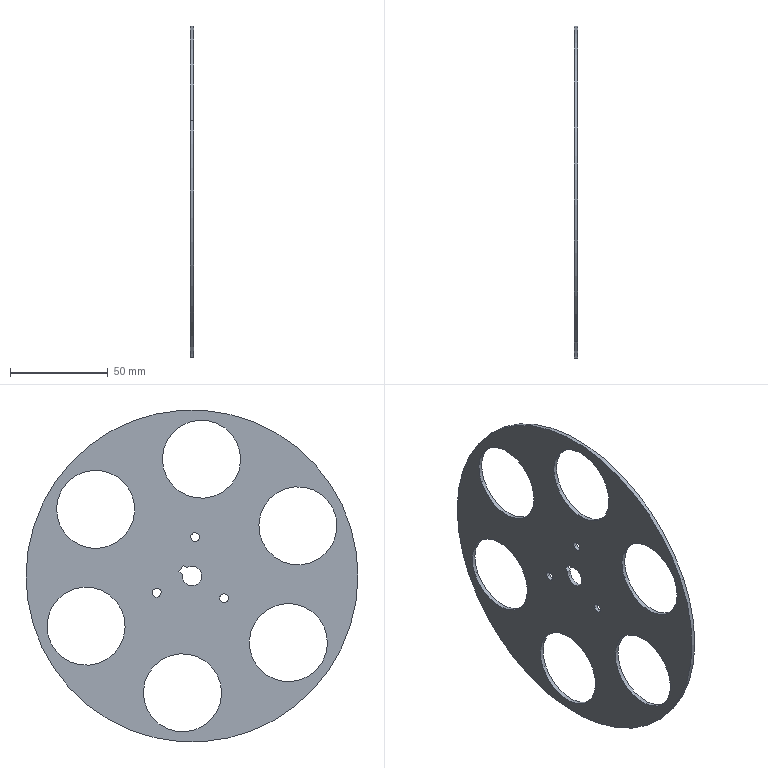Component | SolidWorks | 2018SOLIDWORKS1000000501-1 | 1 solid | 28 faces | box 2 x 170 x 170 mm | volume 30046 mm3 | cylinder 23 | plane 5 | commonest cylinder face diameters 40 x12 4.5 x6 10.1 x3 170 x2 | material SKD11 Ejector Pin
build123d program:
from build123d import *

# Parameters (mm, degrees)
SKETCH1_R                  = 85
SKETCH1_R_2                = 5.05
BOSS_EXTRUDE1_DEPTH        = 2
F_4_5_4_5_DIAMETER_HOLE1_D = 4.5
CIRPATTERN1_COUNT          = 3
SKETCH5_R                  = 20
CUT_EXTRUDE1_DEPTH         = 121.225
CIRPATTERN2_COUNT          = 6
CUT_EXTRUDE2_DEPTH         = 121.225


with BuildPart() as part:
    # Sketch1 → Boss-Extrude1 (new body)
    with BuildSketch(Plane.XY):
        Circle(SKETCH1_R)
        Circle(SKETCH1_R_2, mode=Mode.SUBTRACT)
    extrude(amount=BOSS_EXTRUDE1_DEPTH)

    # 4.5 _4.5_ Diameter Hole1 (through all)
    with Locations(Plane(origin=(0, 0, 0), x_dir=(-1, 0, 0), z_dir=(0, 0, -1))):
        with Locations((20, 0)):
            f_4_5_4_5_diameter_hole1 = Hole(F_4_5_4_5_DIAMETER_HOLE1_D / 2)

    # CirPattern1: 4.5 _4.5_ Diameter Hole1 ×3 about axis
    cirpattern1_axis = Axis((0, 0, 0), (0, 0, 1))
    for i in range(1, CIRPATTERN1_COUNT):
        add(f_4_5_4_5_diameter_hole1.rotate(cirpattern1_axis, i * 360 / CIRPATTERN1_COUNT), mode=Mode.SUBTRACT)

    # Sketch5 → Cut-Extrude1 (cut, through all)
    with BuildSketch(Plane(origin=(0, 0, 0), x_dir=(-1, 0, 0), z_dir=(0, 0, -1))):
        with Locations((60, 0)):
            Circle(SKETCH5_R)
    cut_extrude1 = extrude(amount=-CUT_EXTRUDE1_DEPTH, mode=Mode.SUBTRACT)

    # CirPattern2: Cut-Extrude1 ×6 about axis
    cirpattern2_axis = Axis((0, 0, 0), (0, 0, 1))
    for i in range(1, CIRPATTERN2_COUNT):
        add(cut_extrude1.rotate(cirpattern2_axis, i * 360 / CIRPATTERN2_COUNT), mode=Mode.SUBTRACT)

    # Sketch6 → Cut-Extrude2 (cut, through all)
    with BuildSketch(Plane.XY.offset(2)):
        Polygon((-5.132, 4.889), (-3.132, 1.425), (0.3321, 3.425), (-1.668, 6.889), align=None)
    extrude(amount=-CUT_EXTRUDE2_DEPTH, mode=Mode.SUBTRACT)


solid = part.part

# Placed as in the assembly
solid = solid.moved(Location((2.716, -95.825, 207.018), (64.654, -90, 0)))
STEP:
#1=COLOUR_RGB('',0.7922,0.8196,0.9333);
#2=FILL_AREA_STYLE_COLOUR('',#1);
#3=FILL_AREA_STYLE('',(#2));
#4=SURFACE_STYLE_FILL_AREA(#3);
#5=SURFACE_SIDE_STYLE('',(#4));
#6=SURFACE_STYLE_USAGE(.BOTH.,#5);
#7=PRESENTATION_STYLE_ASSIGNMENT((#6));
#8=CARTESIAN_POINT('',(0.0282,-2.541,9.831));
#9=VERTEX_POINT('',#8);
#10=CARTESIAN_POINT('',(0.0282,-1.118,9.156));
#11=VERTEX_POINT('',#10);
#12=CARTESIAN_POINT('',(0.0282,-1.829,9.494));
#13=DIRECTION('',(1.,0.,-0.));
#14=DIRECTION('',(-0.,0.8226,0.5686));
#15=AXIS2_PLACEMENT_3D('',#12,#13,#14);
#16=CIRCLE('',#15,0.7874);
#17=EDGE_CURVE('',#9,#11,#16,.T.);
#18=ORIENTED_EDGE('',*,*,#17,.F.);
#19=CARTESIAN_POINT('',(0.1069,-2.541,9.831));
#20=VERTEX_POINT('',#19);
#21=CARTESIAN_POINT('',(0.0282,-2.541,9.831));
#22=DIRECTION('',(1.,0.,-0.));
#23=VECTOR('',#22,39.37);
#24=LINE('',#21,#23);
#25=EDGE_CURVE('',#9,#20,#24,.T.);
#26=ORIENTED_EDGE('',*,*,#25,.T.);
#27=CARTESIAN_POINT('',(0.1069,-1.118,9.156));
#28=VERTEX_POINT('',#27);
#29=CARTESIAN_POINT('',(0.1069,-1.829,9.494));
#30=DIRECTION('',(1.,0.,-0.));
#31=DIRECTION('',(-0.,0.8226,0.5686));
#32=AXIS2_PLACEMENT_3D('',#29,#30,#31);
#33=CIRCLE('',#32,0.7874);
#34=EDGE_CURVE('',#20,#28,#33,.T.);
#35=ORIENTED_EDGE('',*,*,#34,.T.);
#36=CARTESIAN_POINT('',(0.0282,-1.118,9.156));
#37=DIRECTION('',(1.,0.,-0.));
#38=VECTOR('',#37,39.37);
#39=LINE('',#36,#38);
#40=EDGE_CURVE('',#11,#28,#39,.T.);
#41=ORIENTED_EDGE('',*,*,#40,.F.);
#42=EDGE_LOOP('',(#18,#26,#35,#41));
#43=FACE_OUTER_BOUND('',#42,.T.);
#44=CARTESIAN_POINT('',(0.0282,-1.829,9.494));
#45=DIRECTION('',(1.,0.,-0.));
#46=DIRECTION('',(-0.,0.9037,-0.4281));
#47=AXIS2_PLACEMENT_3D('',#44,#45,#46);
#48=CYLINDRICAL_SURFACE('',#47,0.7874);
#49=ADVANCED_FACE('',(#43),#48,.F.);
#50=CARTESIAN_POINT('',(0.0282,-4.676,10.842));
#51=VERTEX_POINT('',#50);
#52=CARTESIAN_POINT('',(0.0282,-3.253,10.168));
#53=VERTEX_POINT('',#52);
#54=CARTESIAN_POINT('',(0.0282,-3.964,10.505));
#55=DIRECTION('',(1.,0.,-0.));
#56=DIRECTION('',(0.,-0.08114,0.9967));
#57=AXIS2_PLACEMENT_3D('',#54,#55,#56);
#58=CIRCLE('',#57,0.7874);
#59=EDGE_CURVE('',#51,#53,#58,.T.);
#60=ORIENTED_EDGE('',*,*,#59,.F.);
#61=CARTESIAN_POINT('',(0.1069,-4.676,10.842));
#62=VERTEX_POINT('',#61);
#63=CARTESIAN_POINT('',(0.0282,-4.676,10.842));
#64=DIRECTION('',(1.,0.,-0.));
#65=VECTOR('',#64,39.37);
#66=LINE('',#63,#65);
#67=EDGE_CURVE('',#51,#62,#66,.T.);
#68=ORIENTED_EDGE('',*,*,#67,.T.);
#69=CARTESIAN_POINT('',(0.1069,-3.253,10.168));
#70=VERTEX_POINT('',#69);
#71=CARTESIAN_POINT('',(0.1069,-3.964,10.505));
#72=DIRECTION('',(1.,0.,-0.));
#73=DIRECTION('',(0.,-0.08114,0.9967));
#74=AXIS2_PLACEMENT_3D('',#71,#72,#73);
#75=CIRCLE('',#74,0.7874);
#76=EDGE_CURVE('',#62,#70,#75,.T.);
#77=ORIENTED_EDGE('',*,*,#76,.T.);
#78=CARTESIAN_POINT('',(0.0282,-3.253,10.168));
#79=DIRECTION('',(1.,0.,-0.));
#80=VECTOR('',#79,39.37);
#81=LINE('',#78,#80);
#82=EDGE_CURVE('',#53,#70,#81,.T.);
#83=ORIENTED_EDGE('',*,*,#82,.F.);
#84=EDGE_LOOP('',(#60,#68,#77,#83));
#85=FACE_OUTER_BOUND('',#84,.T.);
#86=CARTESIAN_POINT('',(0.0282,-3.964,10.505));
#87=DIRECTION('',(1.,0.,-0.));
#88=DIRECTION('',(-0.,0.9037,-0.4281));
#89=AXIS2_PLACEMENT_3D('',#86,#87,#88);
#90=CYLINDRICAL_SURFACE('',#89,0.7874);
#91=ADVANCED_FACE('',(#85),#90,.F.);
#92=CARTESIAN_POINT('',(0.0282,-6.619,9.499));
#93=VERTEX_POINT('',#92);
#94=CARTESIAN_POINT('',(0.0282,-5.196,8.824));
#95=VERTEX_POINT('',#94);
#96=CARTESIAN_POINT('',(0.0282,-5.907,9.162));
#97=DIRECTION('',(1.,0.,-0.));
#98=DIRECTION('',(0.,-0.9037,0.4281));
#99=AXIS2_PLACEMENT_3D('',#96,#97,#98);
#100=CIRCLE('',#99,0.7874);
#101=EDGE_CURVE('',#93,#95,#100,.T.);
#102=ORIENTED_EDGE('',*,*,#101,.F.);
#103=CARTESIAN_POINT('',(0.1069,-6.619,9.499));
#104=VERTEX_POINT('',#103);
#105=CARTESIAN_POINT('',(0.0282,-6.619,9.499));
#106=DIRECTION('',(1.,0.,-0.));
#107=VECTOR('',#106,39.37);
#108=LINE('',#105,#107);
#109=EDGE_CURVE('',#93,#104,#108,.T.);
#110=ORIENTED_EDGE('',*,*,#109,.T.);
#111=CARTESIAN_POINT('',(0.1069,-5.196,8.824));
#112=VERTEX_POINT('',#111);
#113=CARTESIAN_POINT('',(0.1069,-5.907,9.162));
#114=DIRECTION('',(1.,0.,-0.));
#115=DIRECTION('',(0.,-0.9037,0.4281));
#116=AXIS2_PLACEMENT_3D('',#113,#114,#115);
#117=CIRCLE('',#116,0.7874);
#118=EDGE_CURVE('',#104,#112,#117,.T.);
#119=ORIENTED_EDGE('',*,*,#118,.T.);
#120=CARTESIAN_POINT('',(0.0282,-5.196,8.824));
#121=DIRECTION('',(1.,0.,-0.));
#122=VECTOR('',#121,39.37);
#123=LINE('',#120,#122);
#124=EDGE_CURVE('',#95,#112,#123,.T.);
#125=ORIENTED_EDGE('',*,*,#124,.F.);
#126=EDGE_LOOP('',(#102,#110,#119,#125));
#127=FACE_OUTER_BOUND('',#126,.T.);
#128=CARTESIAN_POINT('',(0.0282,-5.907,9.162));
#129=DIRECTION('',(1.,0.,-0.));
#130=DIRECTION('',(-0.,0.9037,-0.4281));
#131=AXIS2_PLACEMENT_3D('',#128,#129,#130);
#132=CYLINDRICAL_SURFACE('',#131,0.7874);
#133=ADVANCED_FACE('',(#127),#132,.F.);
#134=CARTESIAN_POINT('',(0.0282,-6.427,7.144));
#135=VERTEX_POINT('',#134);
#136=CARTESIAN_POINT('',(0.0282,-5.004,6.47));
#137=VERTEX_POINT('',#136);
#138=CARTESIAN_POINT('',(0.0282,-5.716,6.807));
#139=DIRECTION('',(1.,0.,-0.));
#140=DIRECTION('',(0.,-0.8226,-0.5686));
#141=AXIS2_PLACEMENT_3D('',#138,#139,#140);
#142=CIRCLE('',#141,0.7874);
#143=EDGE_CURVE('',#135,#137,#142,.T.);
#144=ORIENTED_EDGE('',*,*,#143,.F.);
#145=CARTESIAN_POINT('',(0.1069,-6.427,7.144));
#146=VERTEX_POINT('',#145);
#147=CARTESIAN_POINT('',(0.0282,-6.427,7.144));
#148=DIRECTION('',(1.,0.,-0.));
#149=VECTOR('',#148,39.37);
#150=LINE('',#147,#149);
#151=EDGE_CURVE('',#135,#146,#150,.T.);
#152=ORIENTED_EDGE('',*,*,#151,.T.);
#153=CARTESIAN_POINT('',(0.1069,-5.004,6.47));
#154=VERTEX_POINT('',#153);
#155=CARTESIAN_POINT('',(0.1069,-5.716,6.807));
#156=DIRECTION('',(1.,0.,-0.));
#157=DIRECTION('',(0.,-0.8226,-0.5686));
#158=AXIS2_PLACEMENT_3D('',#155,#156,#157);
#159=CIRCLE('',#158,0.7874);
#160=EDGE_CURVE('',#146,#154,#159,.T.);
#161=ORIENTED_EDGE('',*,*,#160,.T.);
#162=CARTESIAN_POINT('',(0.0282,-5.004,6.47));
#163=DIRECTION('',(1.,0.,-0.));
#164=VECTOR('',#163,39.37);
#165=LINE('',#162,#164);
#166=EDGE_CURVE('',#137,#154,#165,.T.);
#167=ORIENTED_EDGE('',*,*,#166,.F.);
#168=EDGE_LOOP('',(#144,#152,#161,#167));
#169=FACE_OUTER_BOUND('',#168,.T.);
#170=CARTESIAN_POINT('',(0.0282,-5.716,6.807));
#171=DIRECTION('',(1.,0.,-0.));
#172=DIRECTION('',(-0.,0.9037,-0.4281));
#173=AXIS2_PLACEMENT_3D('',#170,#171,#172);
#174=CYLINDRICAL_SURFACE('',#173,0.7874);
#175=ADVANCED_FACE('',(#169),#174,.F.);
#176=CARTESIAN_POINT('',(0.0282,-4.293,6.133));
#177=VERTEX_POINT('',#176);
#178=CARTESIAN_POINT('',(0.0282,-2.869,5.459));
#179=VERTEX_POINT('',#178);
#180=CARTESIAN_POINT('',(0.0282,-3.581,5.796));
#181=DIRECTION('',(1.,0.,-0.));
#182=DIRECTION('',(-0.,0.08114,-0.9967));
#183=AXIS2_PLACEMENT_3D('',#180,#181,#182);
#184=CIRCLE('',#183,0.7874);
#185=EDGE_CURVE('',#177,#179,#184,.T.);
#186=ORIENTED_EDGE('',*,*,#185,.F.);
#187=CARTESIAN_POINT('',(0.1069,-4.293,6.133));
#188=VERTEX_POINT('',#187);
#189=CARTESIAN_POINT('',(0.0282,-4.293,6.133));
#190=DIRECTION('',(1.,0.,-0.));
#191=VECTOR('',#190,39.37);
#192=LINE('',#189,#191);
#193=EDGE_CURVE('',#177,#188,#192,.T.);
#194=ORIENTED_EDGE('',*,*,#193,.T.);
#195=CARTESIAN_POINT('',(0.1069,-2.869,5.459));
#196=VERTEX_POINT('',#195);
#197=CARTESIAN_POINT('',(0.1069,-3.581,5.796));
#198=DIRECTION('',(1.,0.,-0.));
#199=DIRECTION('',(-0.,0.08114,-0.9967));
#200=AXIS2_PLACEMENT_3D('',#197,#198,#199);
#201=CIRCLE('',#200,0.7874);
#202=EDGE_CURVE('',#188,#196,#201,.T.);
#203=ORIENTED_EDGE('',*,*,#202,.T.);
#204=CARTESIAN_POINT('',(0.0282,-2.869,5.459));
#205=DIRECTION('',(1.,0.,-0.));
#206=VECTOR('',#205,39.37);
#207=LINE('',#204,#206);
#208=EDGE_CURVE('',#179,#196,#207,.T.);
#209=ORIENTED_EDGE('',*,*,#208,.F.);
#210=EDGE_LOOP('',(#186,#194,#203,#209));
#211=FACE_OUTER_BOUND('',#210,.T.);
#212=CARTESIAN_POINT('',(0.0282,-3.581,5.796));
#213=DIRECTION('',(1.,0.,-0.));
#214=DIRECTION('',(-0.,0.9037,-0.4281));
#215=AXIS2_PLACEMENT_3D('',#212,#213,#214);
#216=CYLINDRICAL_SURFACE('',#215,0.7874);
#217=ADVANCED_FACE('',(#211),#216,.F.);
#218=CARTESIAN_POINT('',(0.0282,-2.349,7.476));
#219=VERTEX_POINT('',#218);
#220=CARTESIAN_POINT('',(0.0282,-0.9262,6.802));
#221=VERTEX_POINT('',#220);
#222=CARTESIAN_POINT('',(0.0282,-1.638,7.139));
#223=DIRECTION('',(1.,0.,-0.));
#224=DIRECTION('',(-0.,0.9037,-0.4281));
#225=AXIS2_PLACEMENT_3D('',#222,#223,#224);
#226=CIRCLE('',#225,0.7874);
#227=EDGE_CURVE('',#219,#221,#226,.T.);
#228=ORIENTED_EDGE('',*,*,#227,.F.);
#229=CARTESIAN_POINT('',(0.1069,-2.349,7.476));
#230=VERTEX_POINT('',#229);
#231=CARTESIAN_POINT('',(0.0282,-2.349,7.476));
#232=DIRECTION('',(1.,0.,-0.));
#233=VECTOR('',#232,39.37);
#234=LINE('',#231,#233);
#235=EDGE_CURVE('',#219,#230,#234,.T.);
#236=ORIENTED_EDGE('',*,*,#235,.T.);
#237=CARTESIAN_POINT('',(0.1069,-0.9262,6.802));
#238=VERTEX_POINT('',#237);
#239=CARTESIAN_POINT('',(0.1069,-1.638,7.139));
#240=DIRECTION('',(1.,0.,-0.));
#241=DIRECTION('',(-0.,0.9037,-0.4281));
#242=AXIS2_PLACEMENT_3D('',#239,#240,#241);
#243=CIRCLE('',#242,0.7874);
#244=EDGE_CURVE('',#230,#238,#243,.T.);
#245=ORIENTED_EDGE('',*,*,#244,.T.);
#246=CARTESIAN_POINT('',(0.0282,-0.9262,6.802));
#247=DIRECTION('',(1.,0.,-0.));
#248=VECTOR('',#247,39.37);
#249=LINE('',#246,#248);
#250=EDGE_CURVE('',#221,#238,#249,.T.);
#251=ORIENTED_EDGE('',*,*,#250,.F.);
#252=EDGE_LOOP('',(#228,#236,#245,#251));
#253=FACE_OUTER_BOUND('',#252,.T.);
#254=CARTESIAN_POINT('',(0.0282,-1.638,7.139));
#255=DIRECTION('',(1.,0.,-0.));
#256=DIRECTION('',(-0.,0.9037,-0.4281));
#257=AXIS2_PLACEMENT_3D('',#254,#255,#256);
#258=CYLINDRICAL_SURFACE('',#257,0.7874);
#259=ADVANCED_FACE('',(#253),#258,.F.);
#260=CARTESIAN_POINT('',(0.0282,-3.917,8.973));
#261=VERTEX_POINT('',#260);
#262=CARTESIAN_POINT('',(0.0282,-3.756,8.897));
#263=VERTEX_POINT('',#262);
#264=CARTESIAN_POINT('',(0.0282,-3.837,8.935));
#265=DIRECTION('',(1.,0.,-0.));
#266=DIRECTION('',(-0.,0.9037,-0.4281));
#267=AXIS2_PLACEMENT_3D('',#264,#265,#266);
#268=CIRCLE('',#267,0.08858);
#269=EDGE_CURVE('',#261,#263,#268,.T.);
#270=ORIENTED_EDGE('',*,*,#269,.F.);
#271=CARTESIAN_POINT('',(0.1069,-3.917,8.973));
#272=VERTEX_POINT('',#271);
#273=CARTESIAN_POINT('',(0.1069,-3.917,8.973));
#274=DIRECTION('',(1.,0.,-0.));
#275=VECTOR('',#274,39.37);
#276=LINE('',#273,#275);
#277=EDGE_CURVE('',#261,#272,#276,.T.);
#278=ORIENTED_EDGE('',*,*,#277,.T.);
#279=CARTESIAN_POINT('',(0.1069,-3.756,8.897));
#280=VERTEX_POINT('',#279);
#281=CARTESIAN_POINT('',(0.1069,-3.837,8.935));
#282=DIRECTION('',(1.,0.,-0.));
#283=DIRECTION('',(-0.,0.9037,-0.4281));
#284=AXIS2_PLACEMENT_3D('',#281,#282,#283);
#285=CIRCLE('',#284,0.08858);
#286=EDGE_CURVE('',#272,#280,#285,.T.);
#287=ORIENTED_EDGE('',*,*,#286,.T.);
#288=CARTESIAN_POINT('',(0.1069,-3.756,8.897));
#289=DIRECTION('',(1.,0.,-0.));
#290=VECTOR('',#289,39.37);
#291=LINE('',#288,#290);
#292=EDGE_CURVE('',#263,#280,#291,.T.);
#293=ORIENTED_EDGE('',*,*,#292,.F.);
#294=EDGE_LOOP('',(#270,#278,#287,#293));
#295=FACE_OUTER_BOUND('',#294,.T.);
#296=CARTESIAN_POINT('',(0.1069,-3.837,8.935));
#297=DIRECTION('',(1.,0.,-0.));
#298=DIRECTION('',(-0.,0.9037,-0.4281));
#299=AXIS2_PLACEMENT_3D('',#296,#297,#298);
#300=CYLINDRICAL_SURFACE('',#299,0.08858);
#301=ADVANCED_FACE('',(#295),#300,.F.);
#302=CARTESIAN_POINT('',(0.0282,-4.5,7.74));
#303=VERTEX_POINT('',#302);
#304=CARTESIAN_POINT('',(0.0282,-4.34,7.665));
#305=VERTEX_POINT('',#304);
#306=CARTESIAN_POINT('',(0.0282,-4.42,7.703));
#307=DIRECTION('',(1.,0.,-0.));
#308=DIRECTION('',(-0.,0.9037,-0.4281));
#309=AXIS2_PLACEMENT_3D('',#306,#307,#308);
#310=CIRCLE('',#309,0.08858);
#311=EDGE_CURVE('',#303,#305,#310,.T.);
#312=ORIENTED_EDGE('',*,*,#311,.F.);
#313=CARTESIAN_POINT('',(0.1069,-4.5,7.74));
#314=VERTEX_POINT('',#313);
#315=CARTESIAN_POINT('',(0.1069,-4.5,7.74));
#316=DIRECTION('',(1.,0.,-0.));
#317=VECTOR('',#316,39.37);
#318=LINE('',#315,#317);
#319=EDGE_CURVE('',#303,#314,#318,.T.);
#320=ORIENTED_EDGE('',*,*,#319,.T.);
#321=CARTESIAN_POINT('',(0.1069,-4.34,7.665));
#322=VERTEX_POINT('',#321);
#323=CARTESIAN_POINT('',(0.1069,-4.42,7.703));
#324=DIRECTION('',(1.,0.,-0.));
#325=DIRECTION('',(-0.,0.9037,-0.4281));
#326=AXIS2_PLACEMENT_3D('',#323,#324,#325);
#327=CIRCLE('',#326,0.08858);
#328=EDGE_CURVE('',#314,#322,#327,.T.);
#329=ORIENTED_EDGE('',*,*,#328,.T.);
#330=CARTESIAN_POINT('',(0.1069,-4.34,7.665));
#331=DIRECTION('',(1.,0.,-0.));
#332=VECTOR('',#331,39.37);
#333=LINE('',#330,#332);
#334=EDGE_CURVE('',#305,#322,#333,.T.);
#335=ORIENTED_EDGE('',*,*,#334,.F.);
#336=EDGE_LOOP('',(#312,#320,#329,#335));
#337=FACE_OUTER_BOUND('',#336,.T.);
#338=CARTESIAN_POINT('',(0.1069,-4.42,7.703));
#339=DIRECTION('',(1.,0.,-0.));
#340=DIRECTION('',(-0.,0.9037,-0.4281));
#341=AXIS2_PLACEMENT_3D('',#338,#339,#340);
#342=CYLINDRICAL_SURFACE('',#341,0.08858);
#343=ADVANCED_FACE('',(#337),#342,.F.);
#344=CARTESIAN_POINT('',(0.0282,-3.141,7.851));
#345=VERTEX_POINT('',#344);
#346=CARTESIAN_POINT('',(0.0282,-2.981,7.775));
#347=VERTEX_POINT('',#346);
#348=CARTESIAN_POINT('',(0.0282,-3.061,7.813));
#349=DIRECTION('',(1.,0.,-0.));
#350=DIRECTION('',(-0.,0.9037,-0.4281));
#351=AXIS2_PLACEMENT_3D('',#348,#349,#350);
#352=CIRCLE('',#351,0.08858);
#353=EDGE_CURVE('',#345,#347,#352,.T.);
#354=ORIENTED_EDGE('',*,*,#353,.F.);
#355=CARTESIAN_POINT('',(0.1069,-3.141,7.851));
#356=VERTEX_POINT('',#355);
#357=CARTESIAN_POINT('',(0.1069,-3.141,7.851));
#358=DIRECTION('',(1.,0.,-0.));
#359=VECTOR('',#358,39.37);
#360=LINE('',#357,#359);
#361=EDGE_CURVE('',#345,#356,#360,.T.);
#362=ORIENTED_EDGE('',*,*,#361,.T.);
#363=CARTESIAN_POINT('',(0.1069,-2.981,7.775));
#364=VERTEX_POINT('',#363);
#365=CARTESIAN_POINT('',(0.1069,-3.061,7.813));
#366=DIRECTION('',(1.,0.,-0.));
#367=DIRECTION('',(-0.,0.9037,-0.4281));
#368=AXIS2_PLACEMENT_3D('',#365,#366,#367);
#369=CIRCLE('',#368,0.08858);
#370=EDGE_CURVE('',#356,#364,#369,.T.);
#371=ORIENTED_EDGE('',*,*,#370,.T.);
#372=CARTESIAN_POINT('',(0.1069,-2.981,7.775));
#373=DIRECTION('',(1.,0.,-0.));
#374=VECTOR('',#373,39.37);
#375=LINE('',#372,#374);
#376=EDGE_CURVE('',#347,#364,#375,.T.);
#377=ORIENTED_EDGE('',*,*,#376,.F.);
#378=EDGE_LOOP('',(#354,#362,#371,#377));
#379=FACE_OUTER_BOUND('',#378,.T.);
#380=CARTESIAN_POINT('',(0.1069,-3.061,7.813));
#381=DIRECTION('',(1.,0.,-0.));
#382=DIRECTION('',(-0.,0.9037,-0.4281));
#383=AXIS2_PLACEMENT_3D('',#380,#381,#382);
#384=CYLINDRICAL_SURFACE('',#383,0.08858);
#385=ADVANCED_FACE('',(#379),#384,.F.);
#386=CARTESIAN_POINT('',(0.0282,-3.593,8.065));
#387=VERTEX_POINT('',#386);
#388=CARTESIAN_POINT('',(0.0282,-3.952,8.235));
#389=VERTEX_POINT('',#388);
#390=CARTESIAN_POINT('',(0.0282,-3.773,8.15));
#391=DIRECTION('',(-1.,-0.,0.));
#392=DIRECTION('',(0.,-0.9037,0.4281));
#393=AXIS2_PLACEMENT_3D('',#390,#391,#392);
#394=CIRCLE('',#393,0.1988);
#395=EDGE_CURVE('',#387,#389,#394,.T.);
#396=ORIENTED_EDGE('',*,*,#395,.T.);
#397=CARTESIAN_POINT('',(0.1069,-3.952,8.235));
#398=VERTEX_POINT('',#397);
#399=CARTESIAN_POINT('',(0.0282,-3.952,8.235));
#400=DIRECTION('',(1.,0.,-0.));
#401=VECTOR('',#400,39.37);
#402=LINE('',#399,#401);
#403=EDGE_CURVE('',#389,#398,#402,.T.);
#404=ORIENTED_EDGE('',*,*,#403,.T.);
#405=CARTESIAN_POINT('',(0.1069,-3.593,8.065));
#406=VERTEX_POINT('',#405);
#407=CARTESIAN_POINT('',(0.1069,-3.773,8.15));
#408=DIRECTION('',(-1.,-0.,0.));
#409=DIRECTION('',(0.,-0.9037,0.4281));
#410=AXIS2_PLACEMENT_3D('',#407,#408,#409);
#411=CIRCLE('',#410,0.1988);
#412=EDGE_CURVE('',#406,#398,#411,.T.);
#413=ORIENTED_EDGE('',*,*,#412,.F.);
#414=CARTESIAN_POINT('',(0.0282,-3.593,8.065));
#415=DIRECTION('',(1.,0.,-0.));
#416=VECTOR('',#415,39.37);
#417=LINE('',#414,#416);
#418=EDGE_CURVE('',#387,#406,#417,.T.);
#419=ORIENTED_EDGE('',*,*,#418,.F.);
#420=EDGE_LOOP('',(#396,#404,#413,#419));
#421=FACE_OUTER_BOUND('',#420,.T.);
#422=CARTESIAN_POINT('',(0.0282,-3.773,8.15));
#423=DIRECTION('',(1.,0.,-0.));
#424=DIRECTION('',(-0.,0.9037,-0.4281));
#425=AXIS2_PLACEMENT_3D('',#422,#423,#424);
#426=CYLINDRICAL_SURFACE('',#425,0.1988);
#427=ADVANCED_FACE('',(#421),#426,.F.);
#428=CARTESIAN_POINT('',(0.0282,-3.578,8.189));
#429=VERTEX_POINT('',#428);
#430=CARTESIAN_POINT('',(0.0282,-3.773,8.15));
#431=DIRECTION('',(-1.,-0.,0.));
#432=DIRECTION('',(0.,-0.9037,0.4281));
#433=AXIS2_PLACEMENT_3D('',#430,#431,#432);
#434=CIRCLE('',#433,0.1988);
#435=EDGE_CURVE('',#429,#387,#434,.T.);
#436=ORIENTED_EDGE('',*,*,#435,.T.);
#437=ORIENTED_EDGE('',*,*,#418,.T.);
#438=CARTESIAN_POINT('',(0.1069,-3.578,8.189));
#439=VERTEX_POINT('',#438);
#440=CARTESIAN_POINT('',(0.1069,-3.773,8.15));
#441=DIRECTION('',(-1.,-0.,0.));
#442=DIRECTION('',(0.,-0.9037,0.4281));
#443=AXIS2_PLACEMENT_3D('',#440,#441,#442);
#444=CIRCLE('',#443,0.1988);
#445=EDGE_CURVE('',#439,#406,#444,.T.);
#446=ORIENTED_EDGE('',*,*,#445,.F.);
#447=CARTESIAN_POINT('',(0.0282,-3.578,8.189));
#448=DIRECTION('',(1.,0.,-0.));
#449=VECTOR('',#448,39.37);
#450=LINE('',#447,#449);
#451=EDGE_CURVE('',#429,#439,#450,.T.);
#452=ORIENTED_EDGE('',*,*,#451,.F.);
#453=EDGE_LOOP('',(#436,#437,#446,#452));
#454=FACE_OUTER_BOUND('',#453,.T.);
#455=CARTESIAN_POINT('',(0.0282,-3.773,8.15));
#456=DIRECTION('',(1.,0.,-0.));
#457=DIRECTION('',(-0.,0.9037,-0.4281));
#458=AXIS2_PLACEMENT_3D('',#455,#456,#457);
#459=CYLINDRICAL_SURFACE('',#458,0.1988);
#460=ADVANCED_FACE('',(#454),#459,.F.);
#461=CARTESIAN_POINT('',(0.0282,-6.797,9.583));
#462=VERTEX_POINT('',#461);
#463=CARTESIAN_POINT('',(0.0282,-0.7483,6.718));
#464=VERTEX_POINT('',#463);
#465=CARTESIAN_POINT('',(0.0282,-3.773,8.15));
#466=DIRECTION('',(-1.,-0.,0.));
#467=DIRECTION('',(0.,-0.9037,0.4281));
#468=AXIS2_PLACEMENT_3D('',#465,#466,#467);
#469=CIRCLE('',#468,3.346);
#470=EDGE_CURVE('',#462,#464,#469,.T.);
#471=ORIENTED_EDGE('',*,*,#470,.F.);
#472=CARTESIAN_POINT('',(0.1069,-6.797,9.583));
#473=VERTEX_POINT('',#472);
#474=CARTESIAN_POINT('',(0.0282,-6.797,9.583));
#475=DIRECTION('',(1.,0.,-0.));
#476=VECTOR('',#475,39.37);
#477=LINE('',#474,#476);
#478=EDGE_CURVE('',#462,#473,#477,.T.);
#479=ORIENTED_EDGE('',*,*,#478,.T.);
#480=CARTESIAN_POINT('',(0.1069,-0.7483,6.718));
#481=VERTEX_POINT('',#480);
#482=CARTESIAN_POINT('',(0.1069,-3.773,8.15));
#483=DIRECTION('',(-1.,-0.,0.));
#484=DIRECTION('',(0.,-0.9037,0.4281));
#485=AXIS2_PLACEMENT_3D('',#482,#483,#484);
#486=CIRCLE('',#485,3.346);
#487=EDGE_CURVE('',#473,#481,#486,.T.);
#488=ORIENTED_EDGE('',*,*,#487,.T.);
#489=CARTESIAN_POINT('',(0.0282,-0.7483,6.718));
#490=DIRECTION('',(1.,0.,-0.));
#491=VECTOR('',#490,39.37);
#492=LINE('',#489,#491);
#493=EDGE_CURVE('',#464,#481,#492,.T.);
#494=ORIENTED_EDGE('',*,*,#493,.F.);
#495=EDGE_LOOP('',(#471,#479,#488,#494));
#496=FACE_OUTER_BOUND('',#495,.T.);
#497=CARTESIAN_POINT('',(0.0282,-3.773,8.15));
#498=DIRECTION('',(1.,0.,-0.));
#499=DIRECTION('',(-0.,0.9037,-0.4281));
#500=AXIS2_PLACEMENT_3D('',#497,#498,#499);
#501=CYLINDRICAL_SURFACE('',#500,3.346);
#502=ADVANCED_FACE('',(#496),#501,.T.);
#503=CARTESIAN_POINT('',(0.0282,-3.667,8.319));
#504=VERTEX_POINT('',#503);
#505=CARTESIAN_POINT('',(0.0282,-3.597,8.367));
#506=VERTEX_POINT('',#505);
#507=CARTESIAN_POINT('',(0.0282,-3.597,8.367));
#508=DIRECTION('',(-0.,0.8226,0.5686));
#509=VECTOR('',#508,39.37);
#510=LINE('',#507,#509);
#511=EDGE_CURVE('',#504,#506,#510,.T.);
#512=ORIENTED_EDGE('',*,*,#511,.F.);
#513=CARTESIAN_POINT('',(0.0282,-3.773,8.15));
#514=DIRECTION('',(-1.,-0.,0.));
#515=DIRECTION('',(0.,-0.9037,0.4281));
#516=AXIS2_PLACEMENT_3D('',#513,#514,#515);
#517=CIRCLE('',#516,0.1988);
#518=EDGE_CURVE('',#389,#504,#517,.T.);
#519=ORIENTED_EDGE('',*,*,#518,.F.);
#520=ORIENTED_EDGE('',*,*,#395,.F.);
#521=ORIENTED_EDGE('',*,*,#435,.F.);
#522=CARTESIAN_POINT('',(0.0282,-3.508,8.238));
#523=VERTEX_POINT('',#522);
#524=CARTESIAN_POINT('',(0.0282,-3.508,8.238));
#525=DIRECTION('',(0.,-0.8226,-0.5686));
#526=VECTOR('',#525,39.37);
#527=LINE('',#524,#526);
#528=EDGE_CURVE('',#523,#429,#527,.T.);
#529=ORIENTED_EDGE('',*,*,#528,.F.);
#530=CARTESIAN_POINT('',(0.0282,-3.508,8.238));
#531=DIRECTION('',(-0.,0.5686,-0.8226));
#532=VECTOR('',#531,39.37);
#533=LINE('',#530,#532);
#534=EDGE_CURVE('',#506,#523,#533,.T.);
#535=ORIENTED_EDGE('',*,*,#534,.F.);
#536=EDGE_LOOP('',(#512,#519,#520,#521,#529,#535));
#537=FACE_BOUND('',#536,.T.);
#538=CARTESIAN_POINT('',(0.0282,-1.829,9.494));
#539=DIRECTION('',(1.,0.,-0.));
#540=DIRECTION('',(-0.,0.8226,0.5686));
#541=AXIS2_PLACEMENT_3D('',#538,#539,#540);
#542=CIRCLE('',#541,0.7874);
#543=EDGE_CURVE('',#11,#9,#542,.T.);
#544=ORIENTED_EDGE('',*,*,#543,.T.);
#545=ORIENTED_EDGE('',*,*,#17,.T.);
#546=EDGE_LOOP('',(#544,#545));
#547=FACE_BOUND('',#546,.T.);
#548=CARTESIAN_POINT('',(0.0282,-3.964,10.505));
#549=DIRECTION('',(1.,0.,-0.));
#550=DIRECTION('',(0.,-0.08114,0.9967));
#551=AXIS2_PLACEMENT_3D('',#548,#549,#550);
#552=CIRCLE('',#551,0.7874);
#553=EDGE_CURVE('',#53,#51,#552,.T.);
#554=ORIENTED_EDGE('',*,*,#553,.T.);
#555=ORIENTED_EDGE('',*,*,#59,.T.);
#556=EDGE_LOOP('',(#554,#555));
#557=FACE_BOUND('',#556,.T.);
#558=CARTESIAN_POINT('',(0.0282,-5.907,9.162));
#559=DIRECTION('',(1.,0.,-0.));
#560=DIRECTION('',(0.,-0.9037,0.4281));
#561=AXIS2_PLACEMENT_3D('',#558,#559,#560);
#562=CIRCLE('',#561,0.7874);
#563=EDGE_CURVE('',#95,#93,#562,.T.);
#564=ORIENTED_EDGE('',*,*,#563,.T.);
#565=ORIENTED_EDGE('',*,*,#101,.T.);
#566=EDGE_LOOP('',(#564,#565));
#567=FACE_BOUND('',#566,.T.);
#568=CARTESIAN_POINT('',(0.0282,-5.716,6.807));
#569=DIRECTION('',(1.,0.,-0.));
#570=DIRECTION('',(0.,-0.8226,-0.5686));
#571=AXIS2_PLACEMENT_3D('',#568,#569,#570);
#572=CIRCLE('',#571,0.7874);
#573=EDGE_CURVE('',#137,#135,#572,.T.);
#574=ORIENTED_EDGE('',*,*,#573,.T.);
#575=ORIENTED_EDGE('',*,*,#143,.T.);
#576=EDGE_LOOP('',(#574,#575));
#577=FACE_BOUND('',#576,.T.);
#578=CARTESIAN_POINT('',(0.0282,-3.581,5.796));
#579=DIRECTION('',(1.,0.,-0.));
#580=DIRECTION('',(-0.,0.08114,-0.9967));
#581=AXIS2_PLACEMENT_3D('',#578,#579,#580);
#582=CIRCLE('',#581,0.7874);
#583=EDGE_CURVE('',#179,#177,#582,.T.);
#584=ORIENTED_EDGE('',*,*,#583,.T.);
#585=ORIENTED_EDGE('',*,*,#185,.T.);
#586=EDGE_LOOP('',(#584,#585));
#587=FACE_BOUND('',#586,.T.);
#588=CARTESIAN_POINT('',(0.0282,-1.638,7.139));
#589=DIRECTION('',(1.,0.,-0.));
#590=DIRECTION('',(-0.,0.9037,-0.4281));
#591=AXIS2_PLACEMENT_3D('',#588,#589,#590);
#592=CIRCLE('',#591,0.7874);
#593=EDGE_CURVE('',#221,#219,#592,.T.);
#594=ORIENTED_EDGE('',*,*,#593,.T.);
#595=ORIENTED_EDGE('',*,*,#227,.T.);
#596=EDGE_LOOP('',(#594,#595));
#597=FACE_BOUND('',#596,.T.);
#598=CARTESIAN_POINT('',(0.0282,-3.837,8.935));
#599=DIRECTION('',(1.,0.,-0.));
#600=DIRECTION('',(-0.,0.9037,-0.4281));
#601=AXIS2_PLACEMENT_3D('',#598,#599,#600);
#602=CIRCLE('',#601,0.08858);
#603=EDGE_CURVE('',#263,#261,#602,.T.);
#604=ORIENTED_EDGE('',*,*,#603,.T.);
#605=ORIENTED_EDGE('',*,*,#269,.T.);
#606=EDGE_LOOP('',(#604,#605));
#607=FACE_BOUND('',#606,.T.);
#608=CARTESIAN_POINT('',(0.0282,-4.42,7.703));
#609=DIRECTION('',(1.,0.,-0.));
#610=DIRECTION('',(-0.,0.9037,-0.4281));
#611=AXIS2_PLACEMENT_3D('',#608,#609,#610);
#612=CIRCLE('',#611,0.08858);
#613=EDGE_CURVE('',#305,#303,#612,.T.);
#614=ORIENTED_EDGE('',*,*,#613,.T.);
#615=ORIENTED_EDGE('',*,*,#311,.T.);
#616=EDGE_LOOP('',(#614,#615));
#617=FACE_BOUND('',#616,.T.);
#618=CARTESIAN_POINT('',(0.0282,-3.061,7.813));
#619=DIRECTION('',(1.,0.,-0.));
#620=DIRECTION('',(-0.,0.9037,-0.4281));
#621=AXIS2_PLACEMENT_3D('',#618,#619,#620);
#622=CIRCLE('',#621,0.08858);
#623=EDGE_CURVE('',#347,#345,#622,.T.);
#624=ORIENTED_EDGE('',*,*,#623,.T.);
#625=ORIENTED_EDGE('',*,*,#353,.T.);
#626=EDGE_LOOP('',(#624,#625));
#627=FACE_BOUND('',#626,.T.);
#628=CARTESIAN_POINT('',(0.0282,-3.773,8.15));
#629=DIRECTION('',(-1.,-0.,0.));
#630=DIRECTION('',(0.,-0.9037,0.4281));
#631=AXIS2_PLACEMENT_3D('',#628,#629,#630);
#632=CIRCLE('',#631,3.346);
#633=EDGE_CURVE('',#464,#462,#632,.T.);
#634=ORIENTED_EDGE('',*,*,#633,.T.);
#635=ORIENTED_EDGE('',*,*,#470,.T.);
#636=EDGE_LOOP('',(#634,#635));
#637=FACE_OUTER_BOUND('',#636,.T.);
#638=CARTESIAN_POINT('',(0.0282,-3.773,8.15));
#639=DIRECTION('',(-1.,-0.,0.));
#640=DIRECTION('',(0.,-0.9037,0.4281));
#641=AXIS2_PLACEMENT_3D('',#638,#639,#640);
#642=PLANE('',#641);
#643=ADVANCED_FACE('',(#537,#547,#557,#567,#577,#587,#597,#607,#617,#627,#637),#642,.T.);
#644=CARTESIAN_POINT('',(0.1069,-1.829,9.494));
#645=DIRECTION('',(1.,0.,-0.));
#646=DIRECTION('',(-0.,0.8226,0.5686));
#647=AXIS2_PLACEMENT_3D('',#644,#645,#646);
#648=CIRCLE('',#647,0.7874);
#649=EDGE_CURVE('',#28,#20,#648,.T.);
#650=ORIENTED_EDGE('',*,*,#649,.F.);
#651=ORIENTED_EDGE('',*,*,#34,.F.);
#652=EDGE_LOOP('',(#650,#651));
#653=FACE_BOUND('',#652,.T.);
#654=CARTESIAN_POINT('',(0.1069,-3.964,10.505));
#655=DIRECTION('',(1.,0.,-0.));
#656=DIRECTION('',(0.,-0.08114,0.9967));
#657=AXIS2_PLACEMENT_3D('',#654,#655,#656);
#658=CIRCLE('',#657,0.7874);
#659=EDGE_CURVE('',#70,#62,#658,.T.);
#660=ORIENTED_EDGE('',*,*,#659,.F.);
#661=ORIENTED_EDGE('',*,*,#76,.F.);
#662=EDGE_LOOP('',(#660,#661));
#663=FACE_BOUND('',#662,.T.);
#664=CARTESIAN_POINT('',(0.1069,-5.907,9.162));
#665=DIRECTION('',(1.,0.,-0.));
#666=DIRECTION('',(0.,-0.9037,0.4281));
#667=AXIS2_PLACEMENT_3D('',#664,#665,#666);
#668=CIRCLE('',#667,0.7874);
#669=EDGE_CURVE('',#112,#104,#668,.T.);
#670=ORIENTED_EDGE('',*,*,#669,.F.);
#671=ORIENTED_EDGE('',*,*,#118,.F.);
#672=EDGE_LOOP('',(#670,#671));
#673=FACE_BOUND('',#672,.T.);
#674=CARTESIAN_POINT('',(0.1069,-5.716,6.807));
#675=DIRECTION('',(1.,0.,-0.));
#676=DIRECTION('',(0.,-0.8226,-0.5686));
#677=AXIS2_PLACEMENT_3D('',#674,#675,#676);
#678=CIRCLE('',#677,0.7874);
#679=EDGE_CURVE('',#154,#146,#678,.T.);
#680=ORIENTED_EDGE('',*,*,#679,.F.);
#681=ORIENTED_EDGE('',*,*,#160,.F.);
#682=EDGE_LOOP('',(#680,#681));
#683=FACE_BOUND('',#682,.T.);
#684=CARTESIAN_POINT('',(0.1069,-3.581,5.796));
#685=DIRECTION('',(1.,0.,-0.));
#686=DIRECTION('',(-0.,0.08114,-0.9967));
#687=AXIS2_PLACEMENT_3D('',#684,#685,#686);
#688=CIRCLE('',#687,0.7874);
#689=EDGE_CURVE('',#196,#188,#688,.T.);
#690=ORIENTED_EDGE('',*,*,#689,.F.);
#691=ORIENTED_EDGE('',*,*,#202,.F.);
#692=EDGE_LOOP('',(#690,#691));
#693=FACE_BOUND('',#692,.T.);
#694=CARTESIAN_POINT('',(0.1069,-1.638,7.139));
#695=DIRECTION('',(1.,0.,-0.));
#696=DIRECTION('',(-0.,0.9037,-0.4281));
#697=AXIS2_PLACEMENT_3D('',#694,#695,#696);
#698=CIRCLE('',#697,0.7874);
#699=EDGE_CURVE('',#238,#230,#698,.T.);
#700=ORIENTED_EDGE('',*,*,#699,.F.);
#701=ORIENTED_EDGE('',*,*,#244,.F.);
#702=EDGE_LOOP('',(#700,#701));
#703=FACE_BOUND('',#702,.T.);
#704=CARTESIAN_POINT('',(0.1069,-3.837,8.935));
#705=DIRECTION('',(1.,0.,-0.));
#706=DIRECTION('',(-0.,0.9037,-0.4281));
#707=AXIS2_PLACEMENT_3D('',#704,#705,#706);
#708=CIRCLE('',#707,0.08858);
#709=EDGE_CURVE('',#280,#272,#708,.T.);
#710=ORIENTED_EDGE('',*,*,#709,.F.);
#711=ORIENTED_EDGE('',*,*,#286,.F.);
#712=EDGE_LOOP('',(#710,#711));
#713=FACE_BOUND('',#712,.T.);
#714=CARTESIAN_POINT('',(0.1069,-4.42,7.703));
#715=DIRECTION('',(1.,0.,-0.));
#716=DIRECTION('',(-0.,0.9037,-0.4281));
#717=AXIS2_PLACEMENT_3D('',#714,#715,#716);
#718=CIRCLE('',#717,0.08858);
#719=EDGE_CURVE('',#322,#314,#718,.T.);
#720=ORIENTED_EDGE('',*,*,#719,.F.);
#721=ORIENTED_EDGE('',*,*,#328,.F.);
#722=EDGE_LOOP('',(#720,#721));
#723=FACE_BOUND('',#722,.T.);
#724=CARTESIAN_POINT('',(0.1069,-3.061,7.813));
#725=DIRECTION('',(1.,0.,-0.));
#726=DIRECTION('',(-0.,0.9037,-0.4281));
#727=AXIS2_PLACEMENT_3D('',#724,#725,#726);
#728=CIRCLE('',#727,0.08858);
#729=EDGE_CURVE('',#364,#356,#728,.T.);
#730=ORIENTED_EDGE('',*,*,#729,.F.);
#731=ORIENTED_EDGE('',*,*,#370,.F.);
#732=EDGE_LOOP('',(#730,#731));
#733=FACE_BOUND('',#732,.T.);
#734=CARTESIAN_POINT('',(0.1069,-3.773,8.15));
#735=DIRECTION('',(-1.,-0.,0.));
#736=DIRECTION('',(0.,-0.9037,0.4281));
#737=AXIS2_PLACEMENT_3D('',#734,#735,#736);
#738=CIRCLE('',#737,3.346);
#739=EDGE_CURVE('',#481,#473,#738,.T.);
#740=ORIENTED_EDGE('',*,*,#739,.F.);
#741=ORIENTED_EDGE('',*,*,#487,.F.);
#742=EDGE_LOOP('',(#740,#741));
#743=FACE_OUTER_BOUND('',#742,.T.);
#744=ORIENTED_EDGE('',*,*,#445,.T.);
#745=ORIENTED_EDGE('',*,*,#412,.T.);
#746=CARTESIAN_POINT('',(0.1069,-3.667,8.319));
#747=VERTEX_POINT('',#746);
#748=CARTESIAN_POINT('',(0.1069,-3.773,8.15));
#749=DIRECTION('',(-1.,-0.,0.));
#750=DIRECTION('',(0.,-0.9037,0.4281));
#751=AXIS2_PLACEMENT_3D('',#748,#749,#750);
#752=CIRCLE('',#751,0.1988);
#753=EDGE_CURVE('',#398,#747,#752,.T.);
#754=ORIENTED_EDGE('',*,*,#753,.T.);
#755=CARTESIAN_POINT('',(0.1069,-3.597,8.367));
#756=VERTEX_POINT('',#755);
#757=CARTESIAN_POINT('',(0.1069,-3.597,8.367));
#758=DIRECTION('',(-0.,0.8226,0.5686));
#759=VECTOR('',#758,39.37);
#760=LINE('',#757,#759);
#761=EDGE_CURVE('',#747,#756,#760,.T.);
#762=ORIENTED_EDGE('',*,*,#761,.T.);
#763=CARTESIAN_POINT('',(0.1069,-3.508,8.238));
#764=VERTEX_POINT('',#763);
#765=CARTESIAN_POINT('',(0.1069,-3.508,8.238));
#766=DIRECTION('',(-0.,0.5686,-0.8226));
#767=VECTOR('',#766,39.37);
#768=LINE('',#765,#767);
#769=EDGE_CURVE('',#756,#764,#768,.T.);
#770=ORIENTED_EDGE('',*,*,#769,.T.);
#771=CARTESIAN_POINT('',(0.1069,-3.508,8.238));
#772=DIRECTION('',(0.,-0.8226,-0.5686));
#773=VECTOR('',#772,39.37);
#774=LINE('',#771,#773);
#775=EDGE_CURVE('',#764,#439,#774,.T.);
#776=ORIENTED_EDGE('',*,*,#775,.T.);
#777=EDGE_LOOP('',(#744,#745,#754,#762,#770,#776));
#778=FACE_BOUND('',#777,.T.);
#779=CARTESIAN_POINT('',(0.1069,-3.773,8.15));
#780=DIRECTION('',(-1.,-0.,0.));
#781=DIRECTION('',(0.,-0.9037,0.4281));
#782=AXIS2_PLACEMENT_3D('',#779,#780,#781);
#783=PLANE('',#782);
#784=ADVANCED_FACE('',(#653,#663,#673,#683,#693,#703,#713,#723,#733,#743,#778),#783,.F.);
#785=ORIENTED_EDGE('',*,*,#478,.F.);
#786=ORIENTED_EDGE('',*,*,#633,.F.);
#787=ORIENTED_EDGE('',*,*,#493,.T.);
#788=ORIENTED_EDGE('',*,*,#739,.T.);
#789=EDGE_LOOP('',(#785,#786,#787,#788));
#790=FACE_OUTER_BOUND('',#789,.T.);
#791=CARTESIAN_POINT('',(0.0282,-3.773,8.15));
#792=DIRECTION('',(1.,0.,-0.));
#793=DIRECTION('',(-0.,0.9037,-0.4281));
#794=AXIS2_PLACEMENT_3D('',#791,#792,#793);
#795=CYLINDRICAL_SURFACE('',#794,3.346);
#796=ADVANCED_FACE('',(#790),#795,.T.);
#797=ORIENTED_EDGE('',*,*,#403,.F.);
#798=ORIENTED_EDGE('',*,*,#518,.T.);
#799=CARTESIAN_POINT('',(0.0282,-3.667,8.319));
#800=DIRECTION('',(-1.,-0.,0.));
#801=VECTOR('',#800,39.37);
#802=LINE('',#799,#801);
#803=EDGE_CURVE('',#747,#504,#802,.T.);
#804=ORIENTED_EDGE('',*,*,#803,.F.);
#805=ORIENTED_EDGE('',*,*,#753,.F.);
#806=EDGE_LOOP('',(#797,#798,#804,#805));
#807=FACE_OUTER_BOUND('',#806,.T.);
#808=CARTESIAN_POINT('',(0.0282,-3.773,8.15));
#809=DIRECTION('',(1.,0.,-0.));
#810=DIRECTION('',(-0.,0.9037,-0.4281));
#811=AXIS2_PLACEMENT_3D('',#808,#809,#810);
#812=CYLINDRICAL_SURFACE('',#811,0.1988);
#813=ADVANCED_FACE('',(#807),#812,.F.);
#814=ORIENTED_EDGE('',*,*,#361,.F.);
#815=ORIENTED_EDGE('',*,*,#623,.F.);
#816=ORIENTED_EDGE('',*,*,#376,.T.);
#817=ORIENTED_EDGE('',*,*,#729,.T.);
#818=EDGE_LOOP('',(#814,#815,#816,#817));
#819=FACE_OUTER_BOUND('',#818,.T.);
#820=CARTESIAN_POINT('',(0.1069,-3.061,7.813));
#821=DIRECTION('',(1.,0.,-0.));
#822=DIRECTION('',(-0.,0.9037,-0.4281));
#823=AXIS2_PLACEMENT_3D('',#820,#821,#822);
#824=CYLINDRICAL_SURFACE('',#823,0.08858);
#825=ADVANCED_FACE('',(#819),#824,.F.);
#826=ORIENTED_EDGE('',*,*,#319,.F.);
#827=ORIENTED_EDGE('',*,*,#613,.F.);
#828=ORIENTED_EDGE('',*,*,#334,.T.);
#829=ORIENTED_EDGE('',*,*,#719,.T.);
#830=EDGE_LOOP('',(#826,#827,#828,#829));
#831=FACE_OUTER_BOUND('',#830,.T.);
#832=CARTESIAN_POINT('',(0.1069,-4.42,7.703));
#833=DIRECTION('',(1.,0.,-0.));
#834=DIRECTION('',(-0.,0.9037,-0.4281));
#835=AXIS2_PLACEMENT_3D('',#832,#833,#834);
#836=CYLINDRICAL_SURFACE('',#835,0.08858);
#837=ADVANCED_FACE('',(#831),#836,.F.);
#838=ORIENTED_EDGE('',*,*,#277,.F.);
#839=ORIENTED_EDGE('',*,*,#603,.F.);
#840=ORIENTED_EDGE('',*,*,#292,.T.);
#841=ORIENTED_EDGE('',*,*,#709,.T.);
#842=EDGE_LOOP('',(#838,#839,#840,#841));
#843=FACE_OUTER_BOUND('',#842,.T.);
#844=CARTESIAN_POINT('',(0.1069,-3.837,8.935));
#845=DIRECTION('',(1.,0.,-0.));
#846=DIRECTION('',(-0.,0.9037,-0.4281));
#847=AXIS2_PLACEMENT_3D('',#844,#845,#846);
#848=CYLINDRICAL_SURFACE('',#847,0.08858);
#849=ADVANCED_FACE('',(#843),#848,.F.);
#850=ORIENTED_EDGE('',*,*,#235,.F.);
#851=ORIENTED_EDGE('',*,*,#593,.F.);
#852=ORIENTED_EDGE('',*,*,#250,.T.);
#853=ORIENTED_EDGE('',*,*,#699,.T.);
#854=EDGE_LOOP('',(#850,#851,#852,#853));
#855=FACE_OUTER_BOUND('',#854,.T.);
#856=CARTESIAN_POINT('',(0.0282,-1.638,7.139));
#857=DIRECTION('',(1.,0.,-0.));
#858=DIRECTION('',(-0.,0.9037,-0.4281));
#859=AXIS2_PLACEMENT_3D('',#856,#857,#858);
#860=CYLINDRICAL_SURFACE('',#859,0.7874);
#861=ADVANCED_FACE('',(#855),#860,.F.);
#862=ORIENTED_EDGE('',*,*,#193,.F.);
#863=ORIENTED_EDGE('',*,*,#583,.F.);
#864=ORIENTED_EDGE('',*,*,#208,.T.);
#865=ORIENTED_EDGE('',*,*,#689,.T.);
#866=EDGE_LOOP('',(#862,#863,#864,#865));
#867=FACE_OUTER_BOUND('',#866,.T.);
#868=CARTESIAN_POINT('',(0.0282,-3.581,5.796));
#869=DIRECTION('',(1.,0.,-0.));
#870=DIRECTION('',(-0.,0.9037,-0.4281));
#871=AXIS2_PLACEMENT_3D('',#868,#869,#870);
#872=CYLINDRICAL_SURFACE('',#871,0.7874);
#873=ADVANCED_FACE('',(#867),#872,.F.);
#874=ORIENTED_EDGE('',*,*,#151,.F.);
#875=ORIENTED_EDGE('',*,*,#573,.F.);
#876=ORIENTED_EDGE('',*,*,#166,.T.);
#877=ORIENTED_EDGE('',*,*,#679,.T.);
#878=EDGE_LOOP('',(#874,#875,#876,#877));
#879=FACE_OUTER_BOUND('',#878,.T.);
#880=CARTESIAN_POINT('',(0.0282,-5.716,6.807));
#881=DIRECTION('',(1.,0.,-0.));
#882=DIRECTION('',(-0.,0.9037,-0.4281));
#883=AXIS2_PLACEMENT_3D('',#880,#881,#882);
#884=CYLINDRICAL_SURFACE('',#883,0.7874);
#885=ADVANCED_FACE('',(#879),#884,.F.);
#886=ORIENTED_EDGE('',*,*,#109,.F.);
#887=ORIENTED_EDGE('',*,*,#563,.F.);
#888=ORIENTED_EDGE('',*,*,#124,.T.);
#889=ORIENTED_EDGE('',*,*,#669,.T.);
#890=EDGE_LOOP('',(#886,#887,#888,#889));
#891=FACE_OUTER_BOUND('',#890,.T.);
#892=CARTESIAN_POINT('',(0.0282,-5.907,9.162));
#893=DIRECTION('',(1.,0.,-0.));
#894=DIRECTION('',(-0.,0.9037,-0.4281));
#895=AXIS2_PLACEMENT_3D('',#892,#893,#894);
#896=CYLINDRICAL_SURFACE('',#895,0.7874);
#897=ADVANCED_FACE('',(#891),#896,.F.);
#898=ORIENTED_EDGE('',*,*,#67,.F.);
#899=ORIENTED_EDGE('',*,*,#553,.F.);
#900=ORIENTED_EDGE('',*,*,#82,.T.);
#901=ORIENTED_EDGE('',*,*,#659,.T.);
#902=EDGE_LOOP('',(#898,#899,#900,#901));
#903=FACE_OUTER_BOUND('',#902,.T.);
#904=CARTESIAN_POINT('',(0.0282,-3.964,10.505));
#905=DIRECTION('',(1.,0.,-0.));
#906=DIRECTION('',(-0.,0.9037,-0.4281));
#907=AXIS2_PLACEMENT_3D('',#904,#905,#906);
#908=CYLINDRICAL_SURFACE('',#907,0.7874);
#909=ADVANCED_FACE('',(#903),#908,.F.);
#910=ORIENTED_EDGE('',*,*,#25,.F.);
#911=ORIENTED_EDGE('',*,*,#543,.F.);
#912=ORIENTED_EDGE('',*,*,#40,.T.);
#913=ORIENTED_EDGE('',*,*,#649,.T.);
#914=EDGE_LOOP('',(#910,#911,#912,#913));
#915=FACE_OUTER_BOUND('',#914,.T.);
#916=CARTESIAN_POINT('',(0.0282,-1.829,9.494));
#917=DIRECTION('',(1.,0.,-0.));
#918=DIRECTION('',(-0.,0.9037,-0.4281));
#919=AXIS2_PLACEMENT_3D('',#916,#917,#918);
#920=CYLINDRICAL_SURFACE('',#919,0.7874);
#921=ADVANCED_FACE('',(#915),#920,.F.);
#922=ORIENTED_EDGE('',*,*,#534,.T.);
#923=CARTESIAN_POINT('',(0.1069,-3.508,8.238));
#924=DIRECTION('',(-1.,-0.,0.));
#925=VECTOR('',#924,39.37);
#926=LINE('',#923,#925);
#927=EDGE_CURVE('',#764,#523,#926,.T.);
#928=ORIENTED_EDGE('',*,*,#927,.F.);
#929=ORIENTED_EDGE('',*,*,#769,.F.);
#930=CARTESIAN_POINT('',(0.1069,-3.597,8.367));
#931=DIRECTION('',(-1.,-0.,0.));
#932=VECTOR('',#931,39.37);
#933=LINE('',#930,#932);
#934=EDGE_CURVE('',#756,#506,#933,.T.);
#935=ORIENTED_EDGE('',*,*,#934,.T.);
#936=EDGE_LOOP('',(#922,#928,#929,#935));
#937=FACE_OUTER_BOUND('',#936,.T.);
#938=CARTESIAN_POINT('',(0.1069,-3.508,8.238));
#939=DIRECTION('',(-0.,0.8226,0.5686));
#940=DIRECTION('',(-0.,0.5686,-0.8226));
#941=AXIS2_PLACEMENT_3D('',#938,#939,#940);
#942=PLANE('',#941);
#943=ADVANCED_FACE('',(#937),#942,.F.);
#944=ORIENTED_EDGE('',*,*,#803,.T.);
#945=ORIENTED_EDGE('',*,*,#511,.T.);
#946=ORIENTED_EDGE('',*,*,#934,.F.);
#947=ORIENTED_EDGE('',*,*,#761,.F.);
#948=EDGE_LOOP('',(#944,#945,#946,#947));
#949=FACE_OUTER_BOUND('',#948,.T.);
#950=CARTESIAN_POINT('',(0.1069,-3.597,8.367));
#951=DIRECTION('',(0.,-0.5686,0.8226));
#952=DIRECTION('',(-0.,0.8226,0.5686));
#953=AXIS2_PLACEMENT_3D('',#950,#951,#952);
#954=PLANE('',#953);
#955=ADVANCED_FACE('',(#949),#954,.F.);
#956=ORIENTED_EDGE('',*,*,#451,.T.);
#957=ORIENTED_EDGE('',*,*,#775,.F.);
#958=ORIENTED_EDGE('',*,*,#927,.T.);
#959=ORIENTED_EDGE('',*,*,#528,.T.);
#960=EDGE_LOOP('',(#956,#957,#958,#959));
#961=FACE_OUTER_BOUND('',#960,.T.);
#962=CARTESIAN_POINT('',(0.1069,-3.508,8.238));
#963=DIRECTION('',(-0.,0.5686,-0.8226));
#964=DIRECTION('',(0.,-0.8226,-0.5686));
#965=AXIS2_PLACEMENT_3D('',#962,#963,#964);
#966=PLANE('',#965);
#967=ADVANCED_FACE('',(#961),#966,.F.);
#968=CLOSED_SHELL('',(#49,#91,#133,#175,#217,#259,#301,#343,#385,#427,#460,#502,#643,#784,#796,#813,#825,#837,#849,#861,#873,#885,#897,#909,#921,#943,#955,#967));
#969=MANIFOLD_SOLID_BREP('',#968);
#970=STYLED_ITEM('',(#7),#969);
#971=PRESENTATION_LAYER_ASSIGNMENT('','',(#970));
#972=CARTESIAN_POINT('',(0.,0.,0.));
#973=DIRECTION('',(0.,0.,1.));
#974=DIRECTION('',(1.,0.,0.));
#975=AXIS2_PLACEMENT_3D('',#972,#973,#974);
#976=(LENGTH_UNIT()NAMED_UNIT(*)SI_UNIT($,.METRE.));
#977=LENGTH_MEASURE_WITH_UNIT(LENGTH_MEASURE(0.0254),#976);
#978=DIMENSIONAL_EXPONENTS(1.,0.,0.,0.,0.,0.,0.);
#979=(CONVERSION_BASED_UNIT('',#977)LENGTH_UNIT()NAMED_UNIT(#978));
#980=UNCERTAINTY_MEASURE_WITH_UNIT(LENGTH_MEASURE(0.00001),#979,'','');
#981=(NAMED_UNIT(*)PLANE_ANGLE_UNIT()SI_UNIT($,.RADIAN.));
#982=(NAMED_UNIT(*)SI_UNIT($,.STERADIAN.)SOLID_ANGLE_UNIT());
#983=(GEOMETRIC_REPRESENTATION_CONTEXT(3)GLOBAL_UNCERTAINTY_ASSIGNED_CONTEXT((#980))GLOBAL_UNIT_ASSIGNED_CONTEXT((#979,#981,#982))REPRESENTATION_CONTEXT('',''));
#984=ADVANCED_BREP_SHAPE_REPRESENTATION('',(#969,#975),#983);
#985=(LENGTH_UNIT()NAMED_UNIT(*)SI_UNIT($,.METRE.));
#986=LENGTH_MEASURE_WITH_UNIT(LENGTH_MEASURE(0.0254),#985);
#987=DIMENSIONAL_EXPONENTS(1.,0.,0.,0.,0.,0.,0.);
#988=(CONVERSION_BASED_UNIT('',#986)LENGTH_UNIT()NAMED_UNIT(#987));
#989=UNCERTAINTY_MEASURE_WITH_UNIT(LENGTH_MEASURE(0.00001),#988,'','');
#990=(NAMED_UNIT(*)PLANE_ANGLE_UNIT()SI_UNIT($,.RADIAN.));
#991=(NAMED_UNIT(*)SI_UNIT($,.STERADIAN.)SOLID_ANGLE_UNIT());
#992=(GEOMETRIC_REPRESENTATION_CONTEXT(3)GLOBAL_UNCERTAINTY_ASSIGNED_CONTEXT((#989))GLOBAL_UNIT_ASSIGNED_CONTEXT((#988,#990,#991))REPRESENTATION_CONTEXT('',''));
#993=MECHANICAL_DESIGN_GEOMETRIC_PRESENTATION_REPRESENTATION('',(#970),#992);